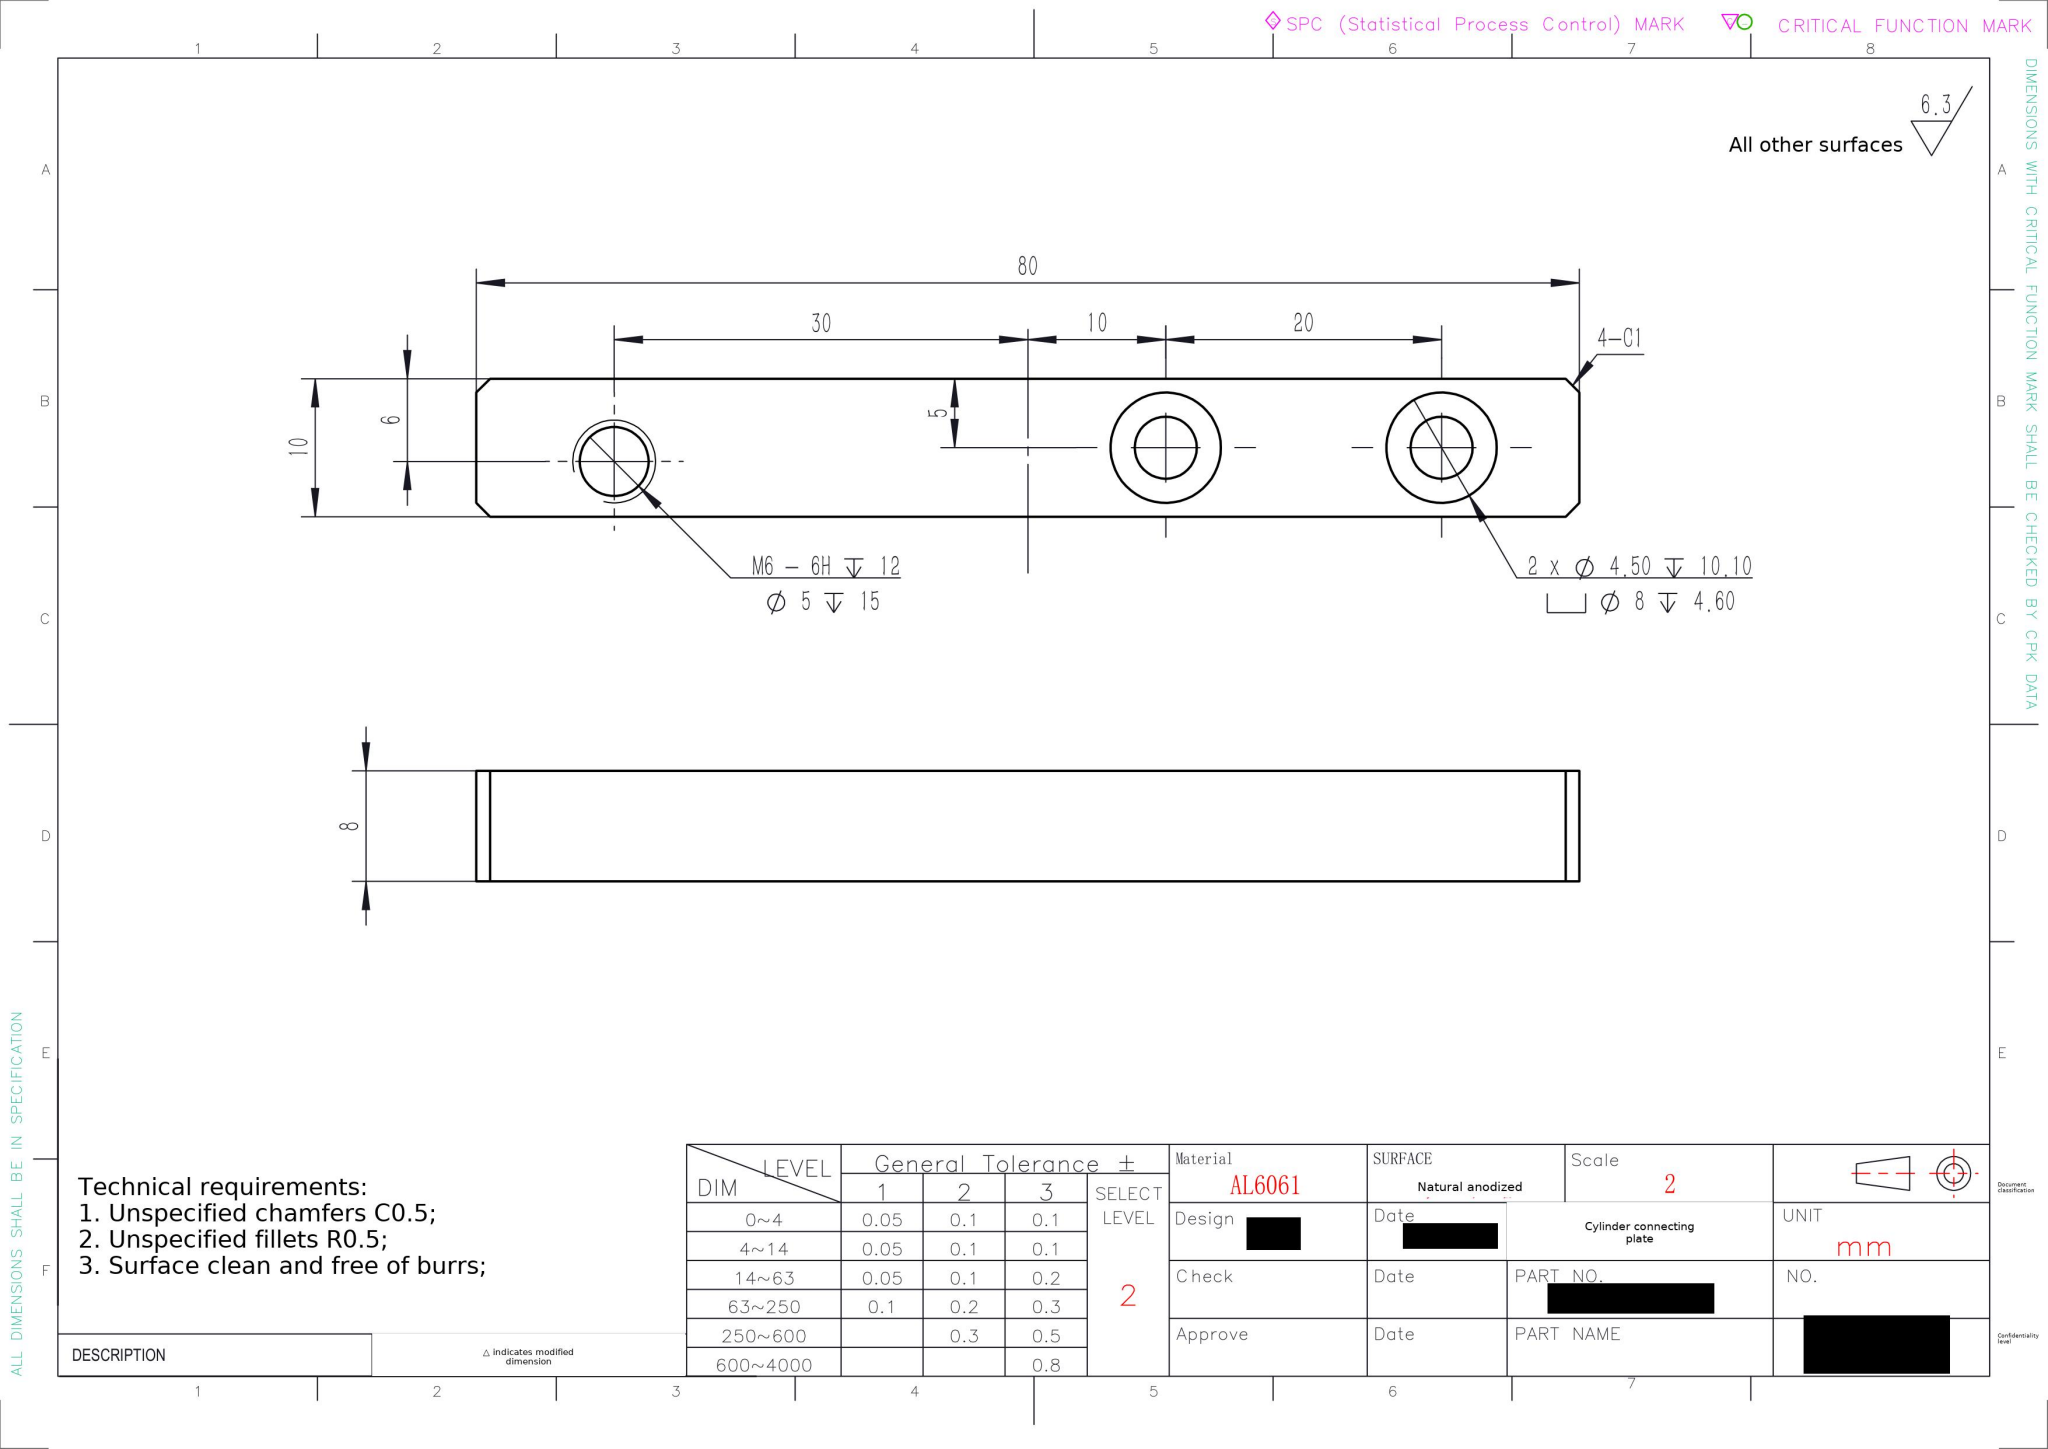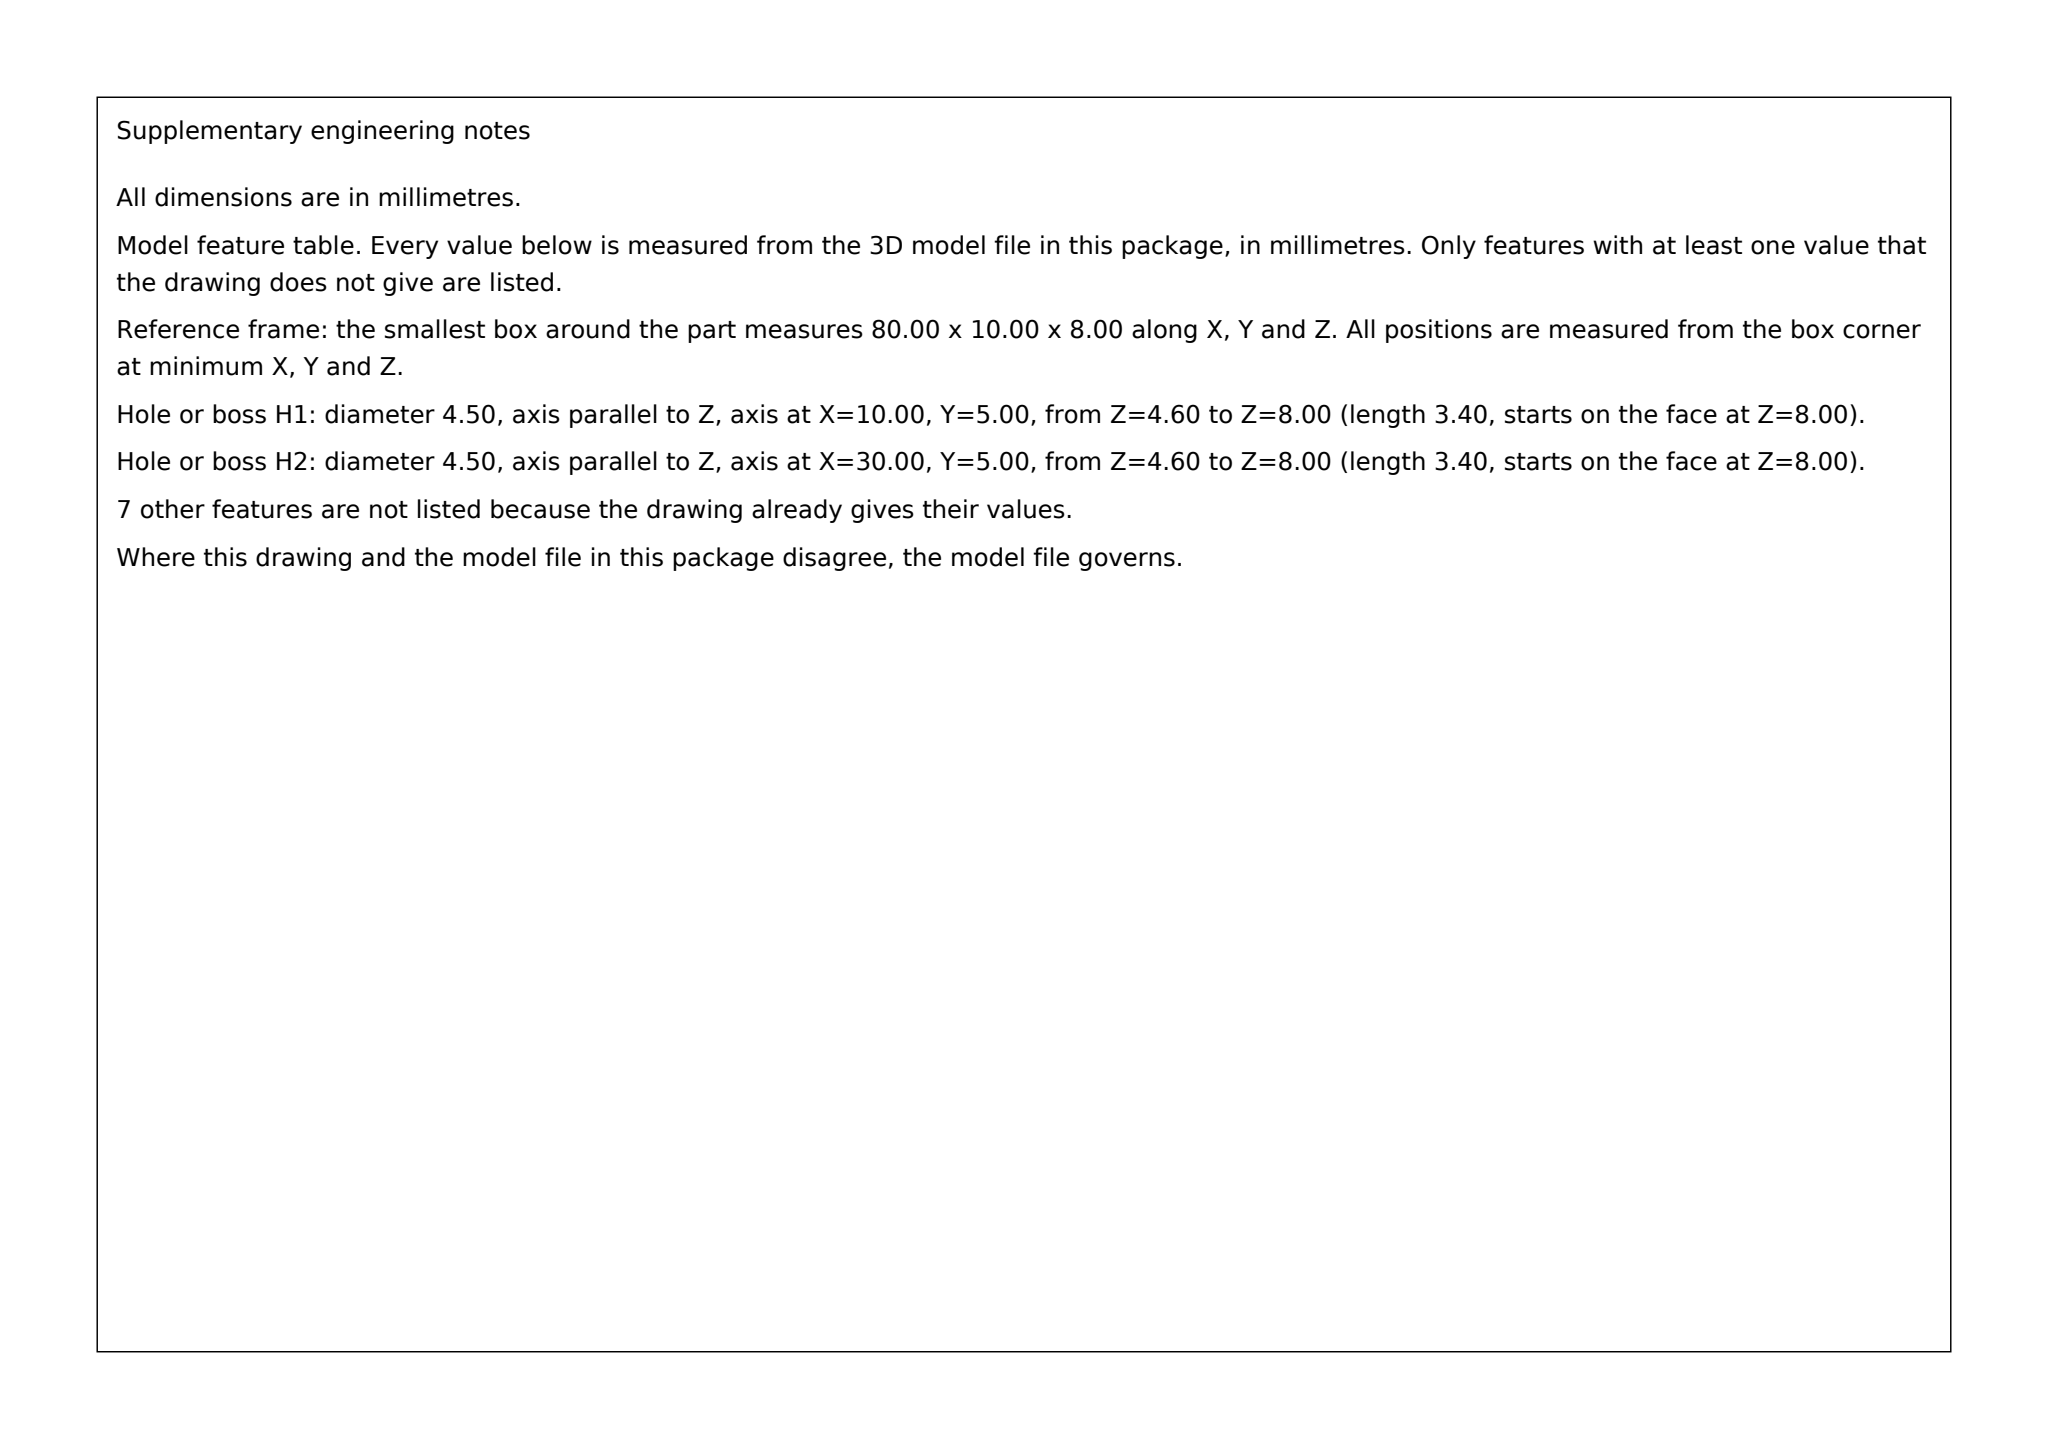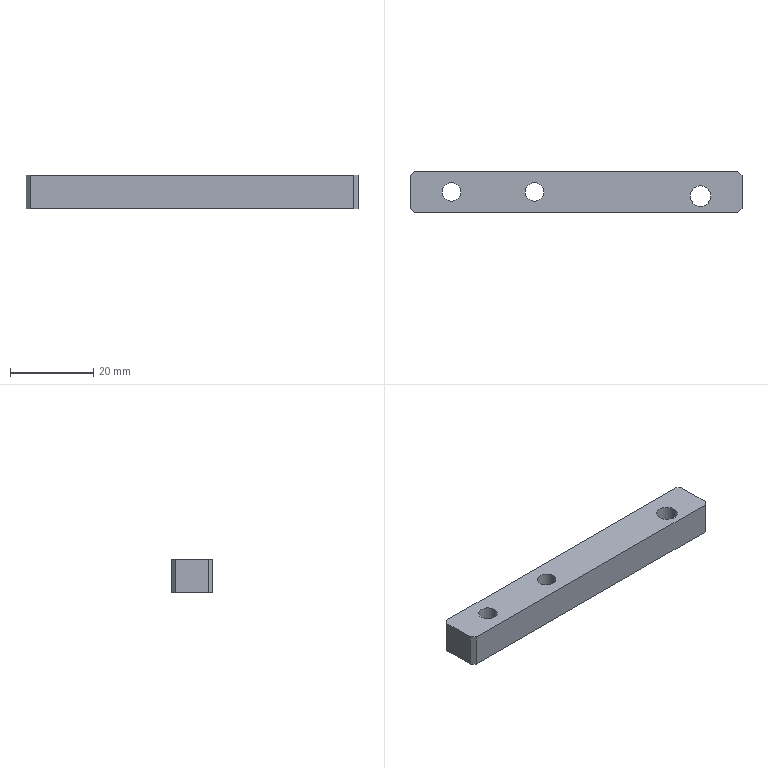Part | SolidWorks | mm | material AL6061 | 1 solid | 22 faces | box 80 x 10 x 8 mm | volume 5656 mm3 | plane 12 | cylinder 10 | commonest cylinder face diameters 8 x4 4.5 x4 5 x2
build123d program:
from build123d import *

# Parameters (mm, degrees)
SKETCH1_W                                         = 80
SKETCH1_H                                         = 10
BOSS_EXTRUDE1_DEPTH                               = 8
CHAMFER1_SIZE                                     = 1
M6_TAPPED_HOLE1_D                                 = 5
M6_TAPPED_HOLE1_DEPTH                             = 15
M6_TAPPED_HOLE1_TIP                               = 1.502
HOLE_SIZE_ACCORDING_TO_TYPE_1_HEXAGON_D           = 4.5
HOLE_SIZE_ACCORDING_TO_TYPE_1_HEXAGON_DEPTH       = 10.1
HOLE_SIZE_ACCORDING_TO_TYPE_1_HEXAGON_CBORE_D     = 8
HOLE_SIZE_ACCORDING_TO_TYPE_1_HEXAGON_CBORE_DEPTH = 4.6
HOLE_SIZE_ACCORDING_TO_TYPE_1_HEXAGON_TIP         = 1.352


with BuildPart() as part:
    # Sketch1 → Boss-Extrude1 (new body)
    with BuildSketch(Plane.XY):
        Rectangle(SKETCH1_W, SKETCH1_H)
    extrude(amount=BOSS_EXTRUDE1_DEPTH)

    # Chamfer1
    chamfer1_edges = [part.edges().sort_by_distance(p)[0] for p in [
        (40, -5, 4),
        (-40, -5, 4),
        (-40, 5, 4),
        (40, 5, 4),
    ]]
    chamfer(chamfer1_edges, length=CHAMFER1_SIZE)

    # M6 Tapped Hole1
    with Locations(Plane.XY.offset(8)):
        with Locations((30, -1)):
            Hole(M6_TAPPED_HOLE1_D / 2, depth=M6_TAPPED_HOLE1_DEPTH)
            with Locations((0, 0, -(M6_TAPPED_HOLE1_DEPTH + M6_TAPPED_HOLE1_TIP / 2))):  # 118° drill point
                Cone(0, M6_TAPPED_HOLE1_D / 2, M6_TAPPED_HOLE1_TIP, mode=Mode.SUBTRACT)

    # Hole Size _ according to_ Type 1 Hexagon
    with Locations(Plane(origin=(0, 0, 0), x_dir=(1, 0, 0), z_dir=(0, 0, -1))):
        with Locations((-10, 0), (-30, 0)):
            CounterBoreHole(HOLE_SIZE_ACCORDING_TO_TYPE_1_HEXAGON_D / 2, HOLE_SIZE_ACCORDING_TO_TYPE_1_HEXAGON_CBORE_D / 2, HOLE_SIZE_ACCORDING_TO_TYPE_1_HEXAGON_CBORE_DEPTH, depth=HOLE_SIZE_ACCORDING_TO_TYPE_1_HEXAGON_DEPTH)
            with Locations((0, 0, -(HOLE_SIZE_ACCORDING_TO_TYPE_1_HEXAGON_DEPTH + HOLE_SIZE_ACCORDING_TO_TYPE_1_HEXAGON_TIP / 2))):  # 118° drill point
                Cone(0, HOLE_SIZE_ACCORDING_TO_TYPE_1_HEXAGON_D / 2, HOLE_SIZE_ACCORDING_TO_TYPE_1_HEXAGON_TIP, mode=Mode.SUBTRACT)


solid = part.part
STEP:
#1=CARTESIAN_POINT('',(-6.,0.,4.6));
#2=VERTEX_POINT('',#1);
#3=CARTESIAN_POINT('',(-14.,0.,4.6));
#4=VERTEX_POINT('',#3);
#5=CARTESIAN_POINT('',(-10.,0.,4.6));
#6=DIRECTION('',(0.,0.,-1.));
#7=DIRECTION('',(-1.,0.,0.));
#8=AXIS2_PLACEMENT_3D('',#5,#6,#7);
#9=CIRCLE('',#8,4.);
#10=EDGE_CURVE('',#2,#4,#9,.T.);
#11=ORIENTED_EDGE('',*,*,#10,.F.);
#12=CARTESIAN_POINT('',(-6.,0.,0.));
#13=VERTEX_POINT('',#12);
#14=CARTESIAN_POINT('',(-6.,0.,0.));
#15=DIRECTION('',(0.,0.,-1.));
#16=VECTOR('',#15,1000.);
#17=LINE('',#14,#16);
#18=EDGE_CURVE('',#2,#13,#17,.T.);
#19=ORIENTED_EDGE('',*,*,#18,.T.);
#20=CARTESIAN_POINT('',(-14.,0.,0.));
#21=VERTEX_POINT('',#20);
#22=CARTESIAN_POINT('',(-10.,0.,0.));
#23=DIRECTION('',(0.,0.,-1.));
#24=DIRECTION('',(-1.,0.,0.));
#25=AXIS2_PLACEMENT_3D('',#22,#23,#24);
#26=CIRCLE('',#25,4.);
#27=EDGE_CURVE('',#13,#21,#26,.T.);
#28=ORIENTED_EDGE('',*,*,#27,.T.);
#29=CARTESIAN_POINT('',(-14.,0.,0.));
#30=DIRECTION('',(0.,0.,-1.));
#31=VECTOR('',#30,1000.);
#32=LINE('',#29,#31);
#33=EDGE_CURVE('',#4,#21,#32,.T.);
#34=ORIENTED_EDGE('',*,*,#33,.F.);
#35=EDGE_LOOP('',(#11,#19,#28,#34));
#36=FACE_OUTER_BOUND('',#35,.T.);
#37=CARTESIAN_POINT('',(-10.,0.,0.));
#38=DIRECTION('',(0.,0.,-1.));
#39=DIRECTION('',(-1.,0.,0.));
#40=AXIS2_PLACEMENT_3D('',#37,#38,#39);
#41=CYLINDRICAL_SURFACE('',#40,4.);
#42=ADVANCED_FACE('',(#36),#41,.F.);
#43=CARTESIAN_POINT('',(-12.25,0.,8.));
#44=VERTEX_POINT('',#43);
#45=CARTESIAN_POINT('',(-7.75,0.,8.));
#46=VERTEX_POINT('',#45);
#47=CARTESIAN_POINT('',(-10.,0.,8.));
#48=DIRECTION('',(0.,0.,1.));
#49=DIRECTION('',(1.,0.,0.));
#50=AXIS2_PLACEMENT_3D('',#47,#48,#49);
#51=CIRCLE('',#50,2.25);
#52=EDGE_CURVE('',#44,#46,#51,.T.);
#53=ORIENTED_EDGE('',*,*,#52,.T.);
#54=CARTESIAN_POINT('',(-7.75,0.,4.6));
#55=VERTEX_POINT('',#54);
#56=CARTESIAN_POINT('',(-7.75,0.,0.));
#57=DIRECTION('',(0.,0.,-1.));
#58=VECTOR('',#57,1000.);
#59=LINE('',#56,#58);
#60=EDGE_CURVE('',#46,#55,#59,.T.);
#61=ORIENTED_EDGE('',*,*,#60,.T.);
#62=CARTESIAN_POINT('',(-12.25,0.,4.6));
#63=VERTEX_POINT('',#62);
#64=CARTESIAN_POINT('',(-10.,0.,4.6));
#65=DIRECTION('',(0.,0.,-1.));
#66=DIRECTION('',(-1.,0.,0.));
#67=AXIS2_PLACEMENT_3D('',#64,#65,#66);
#68=CIRCLE('',#67,2.25);
#69=EDGE_CURVE('',#55,#63,#68,.T.);
#70=ORIENTED_EDGE('',*,*,#69,.T.);
#71=CARTESIAN_POINT('',(-12.25,0.,0.));
#72=DIRECTION('',(0.,0.,-1.));
#73=VECTOR('',#72,1000.);
#74=LINE('',#71,#73);
#75=EDGE_CURVE('',#44,#63,#74,.T.);
#76=ORIENTED_EDGE('',*,*,#75,.F.);
#77=EDGE_LOOP('',(#53,#61,#70,#76));
#78=FACE_OUTER_BOUND('',#77,.T.);
#79=CARTESIAN_POINT('',(-10.,0.,0.));
#80=DIRECTION('',(0.,0.,-1.));
#81=DIRECTION('',(-1.,0.,0.));
#82=AXIS2_PLACEMENT_3D('',#79,#80,#81);
#83=CYLINDRICAL_SURFACE('',#82,2.25);
#84=ADVANCED_FACE('',(#78),#83,.F.);
#85=CARTESIAN_POINT('',(-26.,0.,4.6));
#86=VERTEX_POINT('',#85);
#87=CARTESIAN_POINT('',(-34.,0.,4.6));
#88=VERTEX_POINT('',#87);
#89=CARTESIAN_POINT('',(-30.,0.,4.6));
#90=DIRECTION('',(0.,0.,-1.));
#91=DIRECTION('',(-1.,0.,0.));
#92=AXIS2_PLACEMENT_3D('',#89,#90,#91);
#93=CIRCLE('',#92,4.);
#94=EDGE_CURVE('',#86,#88,#93,.T.);
#95=ORIENTED_EDGE('',*,*,#94,.F.);
#96=CARTESIAN_POINT('',(-26.,0.,0.));
#97=VERTEX_POINT('',#96);
#98=CARTESIAN_POINT('',(-26.,0.,0.));
#99=DIRECTION('',(0.,0.,-1.));
#100=VECTOR('',#99,1000.);
#101=LINE('',#98,#100);
#102=EDGE_CURVE('',#86,#97,#101,.T.);
#103=ORIENTED_EDGE('',*,*,#102,.T.);
#104=CARTESIAN_POINT('',(-34.,0.,0.));
#105=VERTEX_POINT('',#104);
#106=CARTESIAN_POINT('',(-30.,0.,0.));
#107=DIRECTION('',(0.,0.,-1.));
#108=DIRECTION('',(-1.,0.,0.));
#109=AXIS2_PLACEMENT_3D('',#106,#107,#108);
#110=CIRCLE('',#109,4.);
#111=EDGE_CURVE('',#97,#105,#110,.T.);
#112=ORIENTED_EDGE('',*,*,#111,.T.);
#113=CARTESIAN_POINT('',(-34.,0.,0.));
#114=DIRECTION('',(0.,0.,-1.));
#115=VECTOR('',#114,1000.);
#116=LINE('',#113,#115);
#117=EDGE_CURVE('',#88,#105,#116,.T.);
#118=ORIENTED_EDGE('',*,*,#117,.F.);
#119=EDGE_LOOP('',(#95,#103,#112,#118));
#120=FACE_OUTER_BOUND('',#119,.T.);
#121=CARTESIAN_POINT('',(-30.,0.,0.));
#122=DIRECTION('',(0.,0.,-1.));
#123=DIRECTION('',(-1.,0.,0.));
#124=AXIS2_PLACEMENT_3D('',#121,#122,#123);
#125=CYLINDRICAL_SURFACE('',#124,4.);
#126=ADVANCED_FACE('',(#120),#125,.F.);
#127=CARTESIAN_POINT('',(-32.25,0.,8.));
#128=VERTEX_POINT('',#127);
#129=CARTESIAN_POINT('',(-27.75,0.,8.));
#130=VERTEX_POINT('',#129);
#131=CARTESIAN_POINT('',(-30.,0.,8.));
#132=DIRECTION('',(0.,0.,1.));
#133=DIRECTION('',(1.,0.,0.));
#134=AXIS2_PLACEMENT_3D('',#131,#132,#133);
#135=CIRCLE('',#134,2.25);
#136=EDGE_CURVE('',#128,#130,#135,.T.);
#137=ORIENTED_EDGE('',*,*,#136,.T.);
#138=CARTESIAN_POINT('',(-27.75,0.,4.6));
#139=VERTEX_POINT('',#138);
#140=CARTESIAN_POINT('',(-27.75,0.,0.));
#141=DIRECTION('',(0.,0.,-1.));
#142=VECTOR('',#141,1000.);
#143=LINE('',#140,#142);
#144=EDGE_CURVE('',#130,#139,#143,.T.);
#145=ORIENTED_EDGE('',*,*,#144,.T.);
#146=CARTESIAN_POINT('',(-32.25,0.,4.6));
#147=VERTEX_POINT('',#146);
#148=CARTESIAN_POINT('',(-30.,0.,4.6));
#149=DIRECTION('',(0.,0.,-1.));
#150=DIRECTION('',(-1.,0.,0.));
#151=AXIS2_PLACEMENT_3D('',#148,#149,#150);
#152=CIRCLE('',#151,2.25);
#153=EDGE_CURVE('',#139,#147,#152,.T.);
#154=ORIENTED_EDGE('',*,*,#153,.T.);
#155=CARTESIAN_POINT('',(-32.25,0.,0.));
#156=DIRECTION('',(0.,0.,-1.));
#157=VECTOR('',#156,1000.);
#158=LINE('',#155,#157);
#159=EDGE_CURVE('',#128,#147,#158,.T.);
#160=ORIENTED_EDGE('',*,*,#159,.F.);
#161=EDGE_LOOP('',(#137,#145,#154,#160));
#162=FACE_OUTER_BOUND('',#161,.T.);
#163=CARTESIAN_POINT('',(-30.,0.,0.));
#164=DIRECTION('',(0.,0.,-1.));
#165=DIRECTION('',(-1.,0.,0.));
#166=AXIS2_PLACEMENT_3D('',#163,#164,#165);
#167=CYLINDRICAL_SURFACE('',#166,2.25);
#168=ADVANCED_FACE('',(#162),#167,.F.);
#169=CARTESIAN_POINT('',(27.5,-1.,0.));
#170=VERTEX_POINT('',#169);
#171=CARTESIAN_POINT('',(32.5,-1.,0.));
#172=VERTEX_POINT('',#171);
#173=CARTESIAN_POINT('',(30.,-1.,0.));
#174=DIRECTION('',(0.,0.,1.));
#175=DIRECTION('',(1.,0.,0.));
#176=AXIS2_PLACEMENT_3D('',#173,#174,#175);
#177=CIRCLE('',#176,2.5);
#178=EDGE_CURVE('',#170,#172,#177,.T.);
#179=ORIENTED_EDGE('',*,*,#178,.F.);
#180=CARTESIAN_POINT('',(27.5,-1.,8.));
#181=VERTEX_POINT('',#180);
#182=CARTESIAN_POINT('',(27.5,-1.,8.));
#183=DIRECTION('',(0.,0.,1.));
#184=VECTOR('',#183,1000.);
#185=LINE('',#182,#184);
#186=EDGE_CURVE('',#170,#181,#185,.T.);
#187=ORIENTED_EDGE('',*,*,#186,.T.);
#188=CARTESIAN_POINT('',(32.5,-1.,8.));
#189=VERTEX_POINT('',#188);
#190=CARTESIAN_POINT('',(30.,-1.,8.));
#191=DIRECTION('',(0.,0.,1.));
#192=DIRECTION('',(1.,0.,0.));
#193=AXIS2_PLACEMENT_3D('',#190,#191,#192);
#194=CIRCLE('',#193,2.5);
#195=EDGE_CURVE('',#181,#189,#194,.T.);
#196=ORIENTED_EDGE('',*,*,#195,.T.);
#197=CARTESIAN_POINT('',(32.5,-1.,8.));
#198=DIRECTION('',(0.,0.,1.));
#199=VECTOR('',#198,1000.);
#200=LINE('',#197,#199);
#201=EDGE_CURVE('',#172,#189,#200,.T.);
#202=ORIENTED_EDGE('',*,*,#201,.F.);
#203=EDGE_LOOP('',(#179,#187,#196,#202));
#204=FACE_OUTER_BOUND('',#203,.T.);
#205=CARTESIAN_POINT('',(30.,-1.,8.));
#206=DIRECTION('',(0.,0.,1.));
#207=DIRECTION('',(1.,0.,0.));
#208=AXIS2_PLACEMENT_3D('',#205,#206,#207);
#209=CYLINDRICAL_SURFACE('',#208,2.5);
#210=ADVANCED_FACE('',(#204),#209,.F.);
#211=CARTESIAN_POINT('',(40.,-4.,0.));
#212=VERTEX_POINT('',#211);
#213=CARTESIAN_POINT('',(40.,4.,0.));
#214=VERTEX_POINT('',#213);
#215=CARTESIAN_POINT('',(40.,5.,0.));
#216=DIRECTION('',(-0.,1.,0.));
#217=VECTOR('',#216,1000.);
#218=LINE('',#215,#217);
#219=EDGE_CURVE('',#212,#214,#218,.T.);
#220=ORIENTED_EDGE('',*,*,#219,.T.);
#221=CARTESIAN_POINT('',(40.,4.,8.));
#222=VERTEX_POINT('',#221);
#223=CARTESIAN_POINT('',(40.,4.,8.));
#224=DIRECTION('',(0.,0.,1.));
#225=VECTOR('',#224,1000.);
#226=LINE('',#223,#225);
#227=EDGE_CURVE('',#214,#222,#226,.T.);
#228=ORIENTED_EDGE('',*,*,#227,.T.);
#229=CARTESIAN_POINT('',(40.,-4.,8.));
#230=VERTEX_POINT('',#229);
#231=CARTESIAN_POINT('',(40.,5.,8.));
#232=DIRECTION('',(-0.,1.,0.));
#233=VECTOR('',#232,1000.);
#234=LINE('',#231,#233);
#235=EDGE_CURVE('',#230,#222,#234,.T.);
#236=ORIENTED_EDGE('',*,*,#235,.F.);
#237=CARTESIAN_POINT('',(40.,-4.,8.));
#238=DIRECTION('',(0.,0.,-1.));
#239=VECTOR('',#238,1000.);
#240=LINE('',#237,#239);
#241=EDGE_CURVE('',#230,#212,#240,.T.);
#242=ORIENTED_EDGE('',*,*,#241,.T.);
#243=EDGE_LOOP('',(#220,#228,#236,#242));
#244=FACE_OUTER_BOUND('',#243,.T.);
#245=CARTESIAN_POINT('',(40.,5.,8.));
#246=DIRECTION('',(-1.,-0.,0.));
#247=DIRECTION('',(0.,-1.,0.));
#248=AXIS2_PLACEMENT_3D('',#245,#246,#247);
#249=PLANE('',#248);
#250=ADVANCED_FACE('',(#244),#249,.F.);
#251=CARTESIAN_POINT('',(39.,5.,0.));
#252=VERTEX_POINT('',#251);
#253=CARTESIAN_POINT('',(-39.,5.,0.));
#254=VERTEX_POINT('',#253);
#255=CARTESIAN_POINT('',(-40.,5.,0.));
#256=DIRECTION('',(-1.,0.,0.));
#257=VECTOR('',#256,1000.);
#258=LINE('',#255,#257);
#259=EDGE_CURVE('',#252,#254,#258,.T.);
#260=ORIENTED_EDGE('',*,*,#259,.T.);
#261=CARTESIAN_POINT('',(-39.,5.,8.));
#262=VERTEX_POINT('',#261);
#263=CARTESIAN_POINT('',(-39.,5.,8.));
#264=DIRECTION('',(0.,0.,1.));
#265=VECTOR('',#264,1000.);
#266=LINE('',#263,#265);
#267=EDGE_CURVE('',#254,#262,#266,.T.);
#268=ORIENTED_EDGE('',*,*,#267,.T.);
#269=CARTESIAN_POINT('',(39.,5.,8.));
#270=VERTEX_POINT('',#269);
#271=CARTESIAN_POINT('',(-40.,5.,8.));
#272=DIRECTION('',(-1.,0.,0.));
#273=VECTOR('',#272,1000.);
#274=LINE('',#271,#273);
#275=EDGE_CURVE('',#270,#262,#274,.T.);
#276=ORIENTED_EDGE('',*,*,#275,.F.);
#277=CARTESIAN_POINT('',(39.,5.,8.));
#278=DIRECTION('',(0.,0.,-1.));
#279=VECTOR('',#278,1000.);
#280=LINE('',#277,#279);
#281=EDGE_CURVE('',#270,#252,#280,.T.);
#282=ORIENTED_EDGE('',*,*,#281,.T.);
#283=EDGE_LOOP('',(#260,#268,#276,#282));
#284=FACE_OUTER_BOUND('',#283,.T.);
#285=CARTESIAN_POINT('',(-40.,5.,8.));
#286=DIRECTION('',(0.,-1.,0.));
#287=DIRECTION('',(0.,0.,-1.));
#288=AXIS2_PLACEMENT_3D('',#285,#286,#287);
#289=PLANE('',#288);
#290=ADVANCED_FACE('',(#284),#289,.F.);
#291=CARTESIAN_POINT('',(-40.,4.,8.));
#292=VERTEX_POINT('',#291);
#293=CARTESIAN_POINT('',(-40.,-4.,8.));
#294=VERTEX_POINT('',#293);
#295=CARTESIAN_POINT('',(-40.,5.,8.));
#296=DIRECTION('',(0.,-1.,0.));
#297=VECTOR('',#296,1000.);
#298=LINE('',#295,#297);
#299=EDGE_CURVE('',#292,#294,#298,.T.);
#300=ORIENTED_EDGE('',*,*,#299,.F.);
#301=CARTESIAN_POINT('',(-40.,4.,0.));
#302=VERTEX_POINT('',#301);
#303=CARTESIAN_POINT('',(-40.,4.,8.));
#304=DIRECTION('',(0.,0.,-1.));
#305=VECTOR('',#304,1000.);
#306=LINE('',#303,#305);
#307=EDGE_CURVE('',#292,#302,#306,.T.);
#308=ORIENTED_EDGE('',*,*,#307,.T.);
#309=CARTESIAN_POINT('',(-40.,-4.,0.));
#310=VERTEX_POINT('',#309);
#311=CARTESIAN_POINT('',(-40.,5.,0.));
#312=DIRECTION('',(0.,-1.,0.));
#313=VECTOR('',#312,1000.);
#314=LINE('',#311,#313);
#315=EDGE_CURVE('',#302,#310,#314,.T.);
#316=ORIENTED_EDGE('',*,*,#315,.T.);
#317=CARTESIAN_POINT('',(-40.,-4.,8.));
#318=DIRECTION('',(0.,0.,1.));
#319=VECTOR('',#318,1000.);
#320=LINE('',#317,#319);
#321=EDGE_CURVE('',#310,#294,#320,.T.);
#322=ORIENTED_EDGE('',*,*,#321,.T.);
#323=EDGE_LOOP('',(#300,#308,#316,#322));
#324=FACE_OUTER_BOUND('',#323,.T.);
#325=CARTESIAN_POINT('',(-40.,5.,8.));
#326=DIRECTION('',(1.,0.,0.));
#327=DIRECTION('',(0.,0.,-1.));
#328=AXIS2_PLACEMENT_3D('',#325,#326,#327);
#329=PLANE('',#328);
#330=ADVANCED_FACE('',(#324),#329,.F.);
#331=CARTESIAN_POINT('',(-39.,-5.,0.));
#332=VERTEX_POINT('',#331);
#333=CARTESIAN_POINT('',(39.,-5.,0.));
#334=VERTEX_POINT('',#333);
#335=CARTESIAN_POINT('',(-40.,-5.,0.));
#336=DIRECTION('',(1.,0.,0.));
#337=VECTOR('',#336,1000.);
#338=LINE('',#335,#337);
#339=EDGE_CURVE('',#332,#334,#338,.T.);
#340=ORIENTED_EDGE('',*,*,#339,.T.);
#341=CARTESIAN_POINT('',(39.,-5.,8.));
#342=VERTEX_POINT('',#341);
#343=CARTESIAN_POINT('',(39.,-5.,8.));
#344=DIRECTION('',(0.,0.,1.));
#345=VECTOR('',#344,1000.);
#346=LINE('',#343,#345);
#347=EDGE_CURVE('',#334,#342,#346,.T.);
#348=ORIENTED_EDGE('',*,*,#347,.T.);
#349=CARTESIAN_POINT('',(-39.,-5.,8.));
#350=VERTEX_POINT('',#349);
#351=CARTESIAN_POINT('',(-40.,-5.,8.));
#352=DIRECTION('',(1.,0.,0.));
#353=VECTOR('',#352,1000.);
#354=LINE('',#351,#353);
#355=EDGE_CURVE('',#350,#342,#354,.T.);
#356=ORIENTED_EDGE('',*,*,#355,.F.);
#357=CARTESIAN_POINT('',(-39.,-5.,8.));
#358=DIRECTION('',(0.,0.,-1.));
#359=VECTOR('',#358,1000.);
#360=LINE('',#357,#359);
#361=EDGE_CURVE('',#350,#332,#360,.T.);
#362=ORIENTED_EDGE('',*,*,#361,.T.);
#363=EDGE_LOOP('',(#340,#348,#356,#362));
#364=FACE_OUTER_BOUND('',#363,.T.);
#365=CARTESIAN_POINT('',(-40.,-5.,8.));
#366=DIRECTION('',(0.,1.,0.));
#367=DIRECTION('',(0.,0.,1.));
#368=AXIS2_PLACEMENT_3D('',#365,#366,#367);
#369=PLANE('',#368);
#370=ADVANCED_FACE('',(#364),#369,.F.);
#371=ORIENTED_EDGE('',*,*,#52,.F.);
#372=CARTESIAN_POINT('',(-10.,0.,8.));
#373=DIRECTION('',(0.,0.,1.));
#374=DIRECTION('',(1.,0.,0.));
#375=AXIS2_PLACEMENT_3D('',#372,#373,#374);
#376=CIRCLE('',#375,2.25);
#377=EDGE_CURVE('',#46,#44,#376,.T.);
#378=ORIENTED_EDGE('',*,*,#377,.F.);
#379=EDGE_LOOP('',(#371,#378));
#380=FACE_BOUND('',#379,.T.);
#381=ORIENTED_EDGE('',*,*,#136,.F.);
#382=CARTESIAN_POINT('',(-30.,0.,8.));
#383=DIRECTION('',(0.,0.,1.));
#384=DIRECTION('',(1.,0.,0.));
#385=AXIS2_PLACEMENT_3D('',#382,#383,#384);
#386=CIRCLE('',#385,2.25);
#387=EDGE_CURVE('',#130,#128,#386,.T.);
#388=ORIENTED_EDGE('',*,*,#387,.F.);
#389=EDGE_LOOP('',(#381,#388));
#390=FACE_BOUND('',#389,.T.);
#391=CARTESIAN_POINT('',(30.,-1.,8.));
#392=DIRECTION('',(0.,0.,1.));
#393=DIRECTION('',(1.,0.,0.));
#394=AXIS2_PLACEMENT_3D('',#391,#392,#393);
#395=CIRCLE('',#394,2.5);
#396=EDGE_CURVE('',#189,#181,#395,.T.);
#397=ORIENTED_EDGE('',*,*,#396,.F.);
#398=ORIENTED_EDGE('',*,*,#195,.F.);
#399=EDGE_LOOP('',(#397,#398));
#400=FACE_BOUND('',#399,.T.);
#401=ORIENTED_EDGE('',*,*,#275,.T.);
#402=CARTESIAN_POINT('',(-22.,22.,8.));
#403=DIRECTION('',(-0.7071,-0.7071,0.));
#404=VECTOR('',#403,1000.);
#405=LINE('',#402,#404);
#406=EDGE_CURVE('',#262,#292,#405,.T.);
#407=ORIENTED_EDGE('',*,*,#406,.T.);
#408=ORIENTED_EDGE('',*,*,#299,.T.);
#409=CARTESIAN_POINT('',(-22.,-22.,8.));
#410=DIRECTION('',(0.7071,-0.7071,0.));
#411=VECTOR('',#410,1000.);
#412=LINE('',#409,#411);
#413=EDGE_CURVE('',#294,#350,#412,.T.);
#414=ORIENTED_EDGE('',*,*,#413,.T.);
#415=ORIENTED_EDGE('',*,*,#355,.T.);
#416=CARTESIAN_POINT('',(22.,-22.,8.));
#417=DIRECTION('',(0.7071,0.7071,0.));
#418=VECTOR('',#417,1000.);
#419=LINE('',#416,#418);
#420=EDGE_CURVE('',#342,#230,#419,.T.);
#421=ORIENTED_EDGE('',*,*,#420,.T.);
#422=ORIENTED_EDGE('',*,*,#235,.T.);
#423=CARTESIAN_POINT('',(22.,22.,8.));
#424=DIRECTION('',(-0.7071,0.7071,0.));
#425=VECTOR('',#424,1000.);
#426=LINE('',#423,#425);
#427=EDGE_CURVE('',#222,#270,#426,.T.);
#428=ORIENTED_EDGE('',*,*,#427,.T.);
#429=EDGE_LOOP('',(#401,#407,#408,#414,#415,#421,#422,#428));
#430=FACE_OUTER_BOUND('',#429,.T.);
#431=CARTESIAN_POINT('',(0.,0.,8.));
#432=DIRECTION('',(0.,0.,1.));
#433=DIRECTION('',(1.,0.,0.));
#434=AXIS2_PLACEMENT_3D('',#431,#432,#433);
#435=PLANE('',#434);
#436=ADVANCED_FACE('',(#380,#390,#400,#430),#435,.T.);
#437=CARTESIAN_POINT('',(-10.,0.,0.));
#438=DIRECTION('',(0.,0.,-1.));
#439=DIRECTION('',(-1.,0.,0.));
#440=AXIS2_PLACEMENT_3D('',#437,#438,#439);
#441=CIRCLE('',#440,4.);
#442=EDGE_CURVE('',#21,#13,#441,.T.);
#443=ORIENTED_EDGE('',*,*,#442,.F.);
#444=ORIENTED_EDGE('',*,*,#27,.F.);
#445=EDGE_LOOP('',(#443,#444));
#446=FACE_BOUND('',#445,.T.);
#447=CARTESIAN_POINT('',(-30.,0.,0.));
#448=DIRECTION('',(0.,0.,-1.));
#449=DIRECTION('',(-1.,0.,0.));
#450=AXIS2_PLACEMENT_3D('',#447,#448,#449);
#451=CIRCLE('',#450,4.);
#452=EDGE_CURVE('',#105,#97,#451,.T.);
#453=ORIENTED_EDGE('',*,*,#452,.F.);
#454=ORIENTED_EDGE('',*,*,#111,.F.);
#455=EDGE_LOOP('',(#453,#454));
#456=FACE_BOUND('',#455,.T.);
#457=CARTESIAN_POINT('',(30.,-1.,0.));
#458=DIRECTION('',(0.,0.,1.));
#459=DIRECTION('',(1.,0.,0.));
#460=AXIS2_PLACEMENT_3D('',#457,#458,#459);
#461=CIRCLE('',#460,2.5);
#462=EDGE_CURVE('',#172,#170,#461,.T.);
#463=ORIENTED_EDGE('',*,*,#462,.T.);
#464=ORIENTED_EDGE('',*,*,#178,.T.);
#465=EDGE_LOOP('',(#463,#464));
#466=FACE_BOUND('',#465,.T.);
#467=ORIENTED_EDGE('',*,*,#315,.F.);
#468=CARTESIAN_POINT('',(-40.,4.,0.));
#469=DIRECTION('',(0.7071,0.7071,0.));
#470=VECTOR('',#469,1000.);
#471=LINE('',#468,#470);
#472=EDGE_CURVE('',#302,#254,#471,.T.);
#473=ORIENTED_EDGE('',*,*,#472,.T.);
#474=ORIENTED_EDGE('',*,*,#259,.F.);
#475=CARTESIAN_POINT('',(39.,5.,0.));
#476=DIRECTION('',(0.7071,-0.7071,0.));
#477=VECTOR('',#476,1000.);
#478=LINE('',#475,#477);
#479=EDGE_CURVE('',#252,#214,#478,.T.);
#480=ORIENTED_EDGE('',*,*,#479,.T.);
#481=ORIENTED_EDGE('',*,*,#219,.F.);
#482=CARTESIAN_POINT('',(40.,-4.,0.));
#483=DIRECTION('',(-0.7071,-0.7071,0.));
#484=VECTOR('',#483,1000.);
#485=LINE('',#482,#484);
#486=EDGE_CURVE('',#212,#334,#485,.T.);
#487=ORIENTED_EDGE('',*,*,#486,.T.);
#488=ORIENTED_EDGE('',*,*,#339,.F.);
#489=CARTESIAN_POINT('',(-39.,-5.,0.));
#490=DIRECTION('',(-0.7071,0.7071,0.));
#491=VECTOR('',#490,1000.);
#492=LINE('',#489,#491);
#493=EDGE_CURVE('',#332,#310,#492,.T.);
#494=ORIENTED_EDGE('',*,*,#493,.T.);
#495=EDGE_LOOP('',(#467,#473,#474,#480,#481,#487,#488,#494));
#496=FACE_OUTER_BOUND('',#495,.T.);
#497=CARTESIAN_POINT('',(0.,0.,0.));
#498=DIRECTION('',(0.,0.,1.));
#499=DIRECTION('',(1.,0.,0.));
#500=AXIS2_PLACEMENT_3D('',#497,#498,#499);
#501=PLANE('',#500);
#502=ADVANCED_FACE('',(#446,#456,#466,#496),#501,.F.);
#503=ORIENTED_EDGE('',*,*,#406,.F.);
#504=ORIENTED_EDGE('',*,*,#267,.F.);
#505=ORIENTED_EDGE('',*,*,#472,.F.);
#506=ORIENTED_EDGE('',*,*,#307,.F.);
#507=EDGE_LOOP('',(#503,#504,#505,#506));
#508=FACE_OUTER_BOUND('',#507,.T.);
#509=CARTESIAN_POINT('',(-40.,4.,8.));
#510=DIRECTION('',(0.7071,-0.7071,0.));
#511=DIRECTION('',(0.,0.,-1.));
#512=AXIS2_PLACEMENT_3D('',#509,#510,#511);
#513=PLANE('',#512);
#514=ADVANCED_FACE('',(#508),#513,.F.);
#515=ORIENTED_EDGE('',*,*,#427,.F.);
#516=ORIENTED_EDGE('',*,*,#227,.F.);
#517=ORIENTED_EDGE('',*,*,#479,.F.);
#518=ORIENTED_EDGE('',*,*,#281,.F.);
#519=EDGE_LOOP('',(#515,#516,#517,#518));
#520=FACE_OUTER_BOUND('',#519,.T.);
#521=CARTESIAN_POINT('',(39.,5.,8.));
#522=DIRECTION('',(-0.7071,-0.7071,0.));
#523=DIRECTION('',(0.,0.,-1.));
#524=AXIS2_PLACEMENT_3D('',#521,#522,#523);
#525=PLANE('',#524);
#526=ADVANCED_FACE('',(#520),#525,.F.);
#527=ORIENTED_EDGE('',*,*,#420,.F.);
#528=ORIENTED_EDGE('',*,*,#347,.F.);
#529=ORIENTED_EDGE('',*,*,#486,.F.);
#530=ORIENTED_EDGE('',*,*,#241,.F.);
#531=EDGE_LOOP('',(#527,#528,#529,#530));
#532=FACE_OUTER_BOUND('',#531,.T.);
#533=CARTESIAN_POINT('',(40.,-4.,8.));
#534=DIRECTION('',(-0.7071,0.7071,0.));
#535=DIRECTION('',(0.,0.,-1.));
#536=AXIS2_PLACEMENT_3D('',#533,#534,#535);
#537=PLANE('',#536);
#538=ADVANCED_FACE('',(#532),#537,.F.);
#539=ORIENTED_EDGE('',*,*,#413,.F.);
#540=ORIENTED_EDGE('',*,*,#321,.F.);
#541=ORIENTED_EDGE('',*,*,#493,.F.);
#542=ORIENTED_EDGE('',*,*,#361,.F.);
#543=EDGE_LOOP('',(#539,#540,#541,#542));
#544=FACE_OUTER_BOUND('',#543,.T.);
#545=CARTESIAN_POINT('',(-39.,-5.,8.));
#546=DIRECTION('',(0.7071,0.7071,0.));
#547=DIRECTION('',(0.,0.,-1.));
#548=AXIS2_PLACEMENT_3D('',#545,#546,#547);
#549=PLANE('',#548);
#550=ADVANCED_FACE('',(#544),#549,.F.);
#551=ORIENTED_EDGE('',*,*,#186,.F.);
#552=ORIENTED_EDGE('',*,*,#462,.F.);
#553=ORIENTED_EDGE('',*,*,#201,.T.);
#554=ORIENTED_EDGE('',*,*,#396,.T.);
#555=EDGE_LOOP('',(#551,#552,#553,#554));
#556=FACE_OUTER_BOUND('',#555,.T.);
#557=CARTESIAN_POINT('',(30.,-1.,8.));
#558=DIRECTION('',(0.,0.,1.));
#559=DIRECTION('',(1.,0.,0.));
#560=AXIS2_PLACEMENT_3D('',#557,#558,#559);
#561=CYLINDRICAL_SURFACE('',#560,2.5);
#562=ADVANCED_FACE('',(#556),#561,.F.);
#563=ORIENTED_EDGE('',*,*,#144,.F.);
#564=ORIENTED_EDGE('',*,*,#387,.T.);
#565=ORIENTED_EDGE('',*,*,#159,.T.);
#566=CARTESIAN_POINT('',(-30.,0.,4.6));
#567=DIRECTION('',(0.,0.,-1.));
#568=DIRECTION('',(-1.,0.,0.));
#569=AXIS2_PLACEMENT_3D('',#566,#567,#568);
#570=CIRCLE('',#569,2.25);
#571=EDGE_CURVE('',#147,#139,#570,.T.);
#572=ORIENTED_EDGE('',*,*,#571,.T.);
#573=EDGE_LOOP('',(#563,#564,#565,#572));
#574=FACE_OUTER_BOUND('',#573,.T.);
#575=CARTESIAN_POINT('',(-30.,0.,0.));
#576=DIRECTION('',(0.,0.,-1.));
#577=DIRECTION('',(-1.,0.,0.));
#578=AXIS2_PLACEMENT_3D('',#575,#576,#577);
#579=CYLINDRICAL_SURFACE('',#578,2.25);
#580=ADVANCED_FACE('',(#574),#579,.F.);
#581=ORIENTED_EDGE('',*,*,#571,.F.);
#582=ORIENTED_EDGE('',*,*,#153,.F.);
#583=EDGE_LOOP('',(#581,#582));
#584=FACE_BOUND('',#583,.T.);
#585=CARTESIAN_POINT('',(-30.,0.,4.6));
#586=DIRECTION('',(0.,0.,-1.));
#587=DIRECTION('',(-1.,0.,0.));
#588=AXIS2_PLACEMENT_3D('',#585,#586,#587);
#589=CIRCLE('',#588,4.);
#590=EDGE_CURVE('',#88,#86,#589,.T.);
#591=ORIENTED_EDGE('',*,*,#590,.T.);
#592=ORIENTED_EDGE('',*,*,#94,.T.);
#593=EDGE_LOOP('',(#591,#592));
#594=FACE_OUTER_BOUND('',#593,.T.);
#595=CARTESIAN_POINT('',(-27.75,0.,4.6));
#596=DIRECTION('',(0.,0.,1.));
#597=DIRECTION('',(1.,0.,0.));
#598=AXIS2_PLACEMENT_3D('',#595,#596,#597);
#599=PLANE('',#598);
#600=ADVANCED_FACE('',(#584,#594),#599,.F.);
#601=ORIENTED_EDGE('',*,*,#102,.F.);
#602=ORIENTED_EDGE('',*,*,#590,.F.);
#603=ORIENTED_EDGE('',*,*,#117,.T.);
#604=ORIENTED_EDGE('',*,*,#452,.T.);
#605=EDGE_LOOP('',(#601,#602,#603,#604));
#606=FACE_OUTER_BOUND('',#605,.T.);
#607=CARTESIAN_POINT('',(-30.,0.,0.));
#608=DIRECTION('',(0.,0.,-1.));
#609=DIRECTION('',(-1.,0.,0.));
#610=AXIS2_PLACEMENT_3D('',#607,#608,#609);
#611=CYLINDRICAL_SURFACE('',#610,4.);
#612=ADVANCED_FACE('',(#606),#611,.F.);
#613=ORIENTED_EDGE('',*,*,#60,.F.);
#614=ORIENTED_EDGE('',*,*,#377,.T.);
#615=ORIENTED_EDGE('',*,*,#75,.T.);
#616=CARTESIAN_POINT('',(-10.,0.,4.6));
#617=DIRECTION('',(0.,0.,-1.));
#618=DIRECTION('',(-1.,0.,0.));
#619=AXIS2_PLACEMENT_3D('',#616,#617,#618);
#620=CIRCLE('',#619,2.25);
#621=EDGE_CURVE('',#63,#55,#620,.T.);
#622=ORIENTED_EDGE('',*,*,#621,.T.);
#623=EDGE_LOOP('',(#613,#614,#615,#622));
#624=FACE_OUTER_BOUND('',#623,.T.);
#625=CARTESIAN_POINT('',(-10.,0.,0.));
#626=DIRECTION('',(0.,0.,-1.));
#627=DIRECTION('',(-1.,0.,0.));
#628=AXIS2_PLACEMENT_3D('',#625,#626,#627);
#629=CYLINDRICAL_SURFACE('',#628,2.25);
#630=ADVANCED_FACE('',(#624),#629,.F.);
#631=ORIENTED_EDGE('',*,*,#621,.F.);
#632=ORIENTED_EDGE('',*,*,#69,.F.);
#633=EDGE_LOOP('',(#631,#632));
#634=FACE_BOUND('',#633,.T.);
#635=CARTESIAN_POINT('',(-10.,0.,4.6));
#636=DIRECTION('',(0.,0.,-1.));
#637=DIRECTION('',(-1.,0.,0.));
#638=AXIS2_PLACEMENT_3D('',#635,#636,#637);
#639=CIRCLE('',#638,4.);
#640=EDGE_CURVE('',#4,#2,#639,.T.);
#641=ORIENTED_EDGE('',*,*,#640,.T.);
#642=ORIENTED_EDGE('',*,*,#10,.T.);
#643=EDGE_LOOP('',(#641,#642));
#644=FACE_OUTER_BOUND('',#643,.T.);
#645=CARTESIAN_POINT('',(-7.75,0.,4.6));
#646=DIRECTION('',(0.,0.,1.));
#647=DIRECTION('',(1.,0.,0.));
#648=AXIS2_PLACEMENT_3D('',#645,#646,#647);
#649=PLANE('',#648);
#650=ADVANCED_FACE('',(#634,#644),#649,.F.);
#651=ORIENTED_EDGE('',*,*,#18,.F.);
#652=ORIENTED_EDGE('',*,*,#640,.F.);
#653=ORIENTED_EDGE('',*,*,#33,.T.);
#654=ORIENTED_EDGE('',*,*,#442,.T.);
#655=EDGE_LOOP('',(#651,#652,#653,#654));
#656=FACE_OUTER_BOUND('',#655,.T.);
#657=CARTESIAN_POINT('',(-10.,0.,0.));
#658=DIRECTION('',(0.,0.,-1.));
#659=DIRECTION('',(-1.,0.,0.));
#660=AXIS2_PLACEMENT_3D('',#657,#658,#659);
#661=CYLINDRICAL_SURFACE('',#660,4.);
#662=ADVANCED_FACE('',(#656),#661,.F.);
#663=CLOSED_SHELL('',(#42,#84,#126,#168,#210,#250,#290,#330,#370,#436,#502,#514,#526,#538,#550,#562,#580,#600,#612,#630,#650,#662));
#664=MANIFOLD_SOLID_BREP('',#663);
#665=CARTESIAN_POINT('',(0.,0.,0.));
#666=DIRECTION('',(0.,0.,1.));
#667=DIRECTION('',(1.,0.,0.));
#668=AXIS2_PLACEMENT_3D('',#665,#666,#667);
#669=(LENGTH_UNIT()NAMED_UNIT(*)SI_UNIT(.MILLI.,.METRE.));
#670=UNCERTAINTY_MEASURE_WITH_UNIT(LENGTH_MEASURE(0.00001),#669,'','');
#671=(NAMED_UNIT(*)PLANE_ANGLE_UNIT()SI_UNIT($,.RADIAN.));
#672=(NAMED_UNIT(*)SI_UNIT($,.STERADIAN.)SOLID_ANGLE_UNIT());
#673=(GEOMETRIC_REPRESENTATION_CONTEXT(3)GLOBAL_UNCERTAINTY_ASSIGNED_CONTEXT((#670))GLOBAL_UNIT_ASSIGNED_CONTEXT((#669,#671,#672))REPRESENTATION_CONTEXT('',''));
#674=ADVANCED_BREP_SHAPE_REPRESENTATION('',(#664,#668),#673);